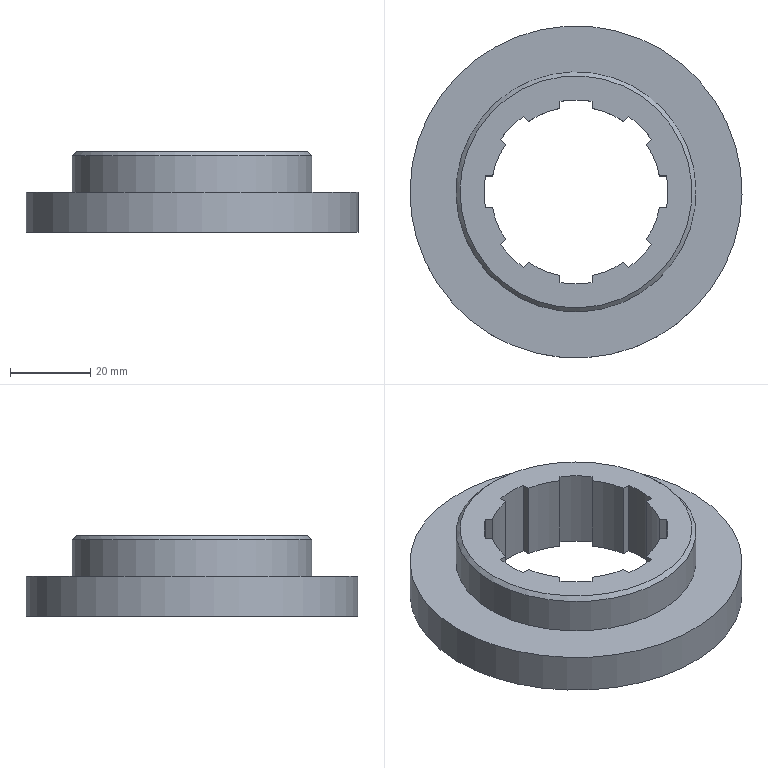Component | NX | ZYC44 | 1 solid | 38 faces | volume 51662 mm3 | plane 19 | cylinder 18 | cone 1 | commonest cylinder face diameters 42.5 x8 46 x8 83 x1 60 x1